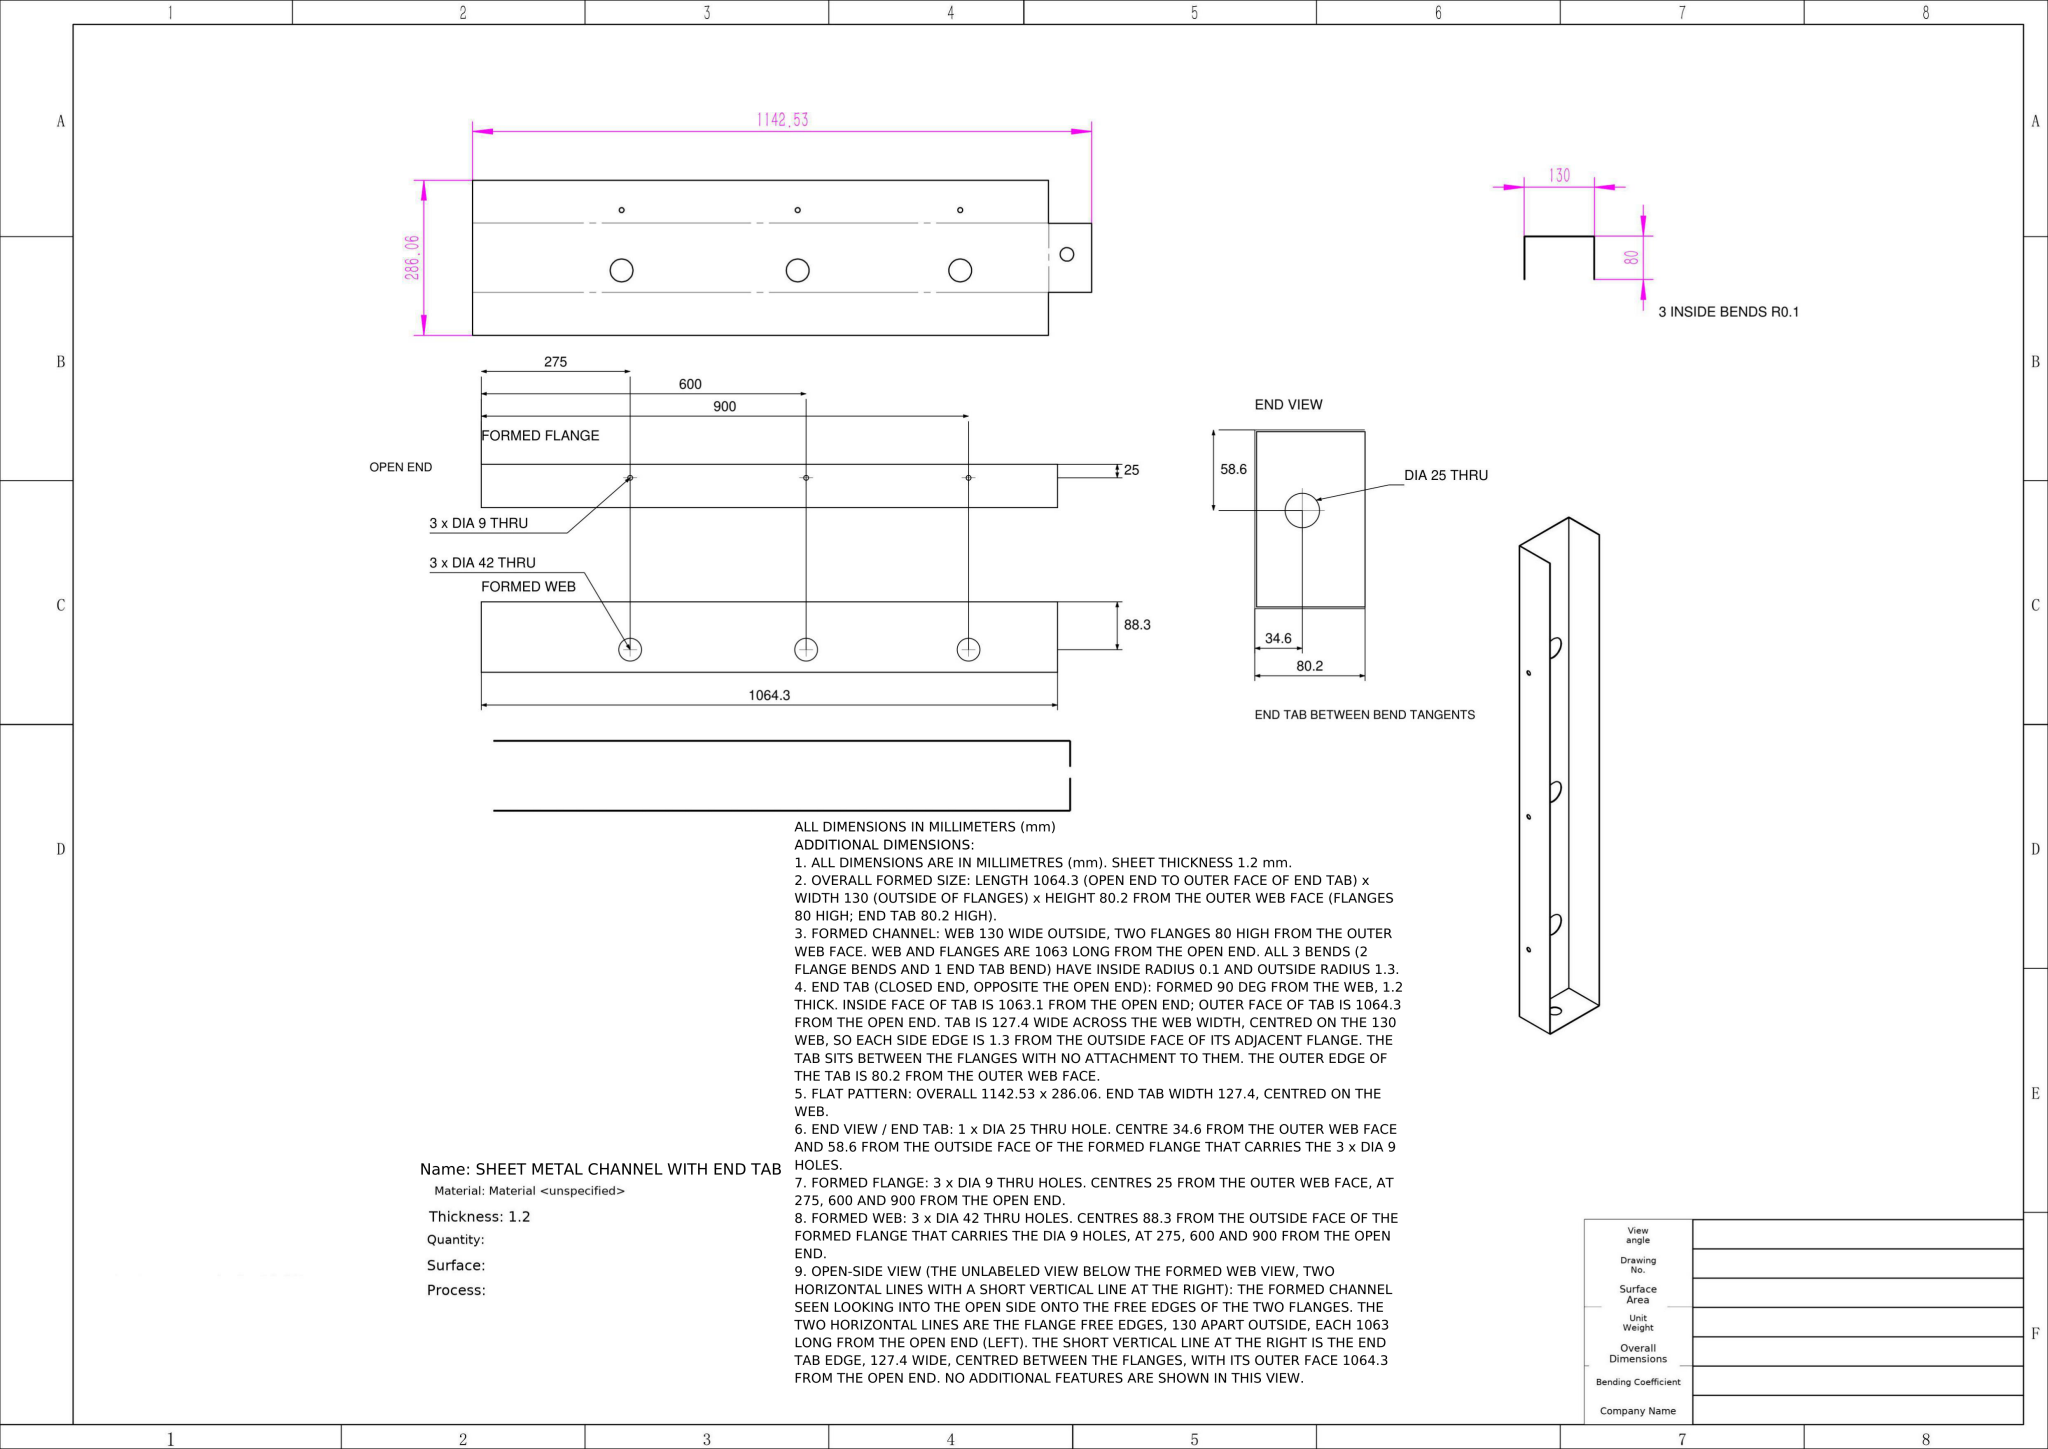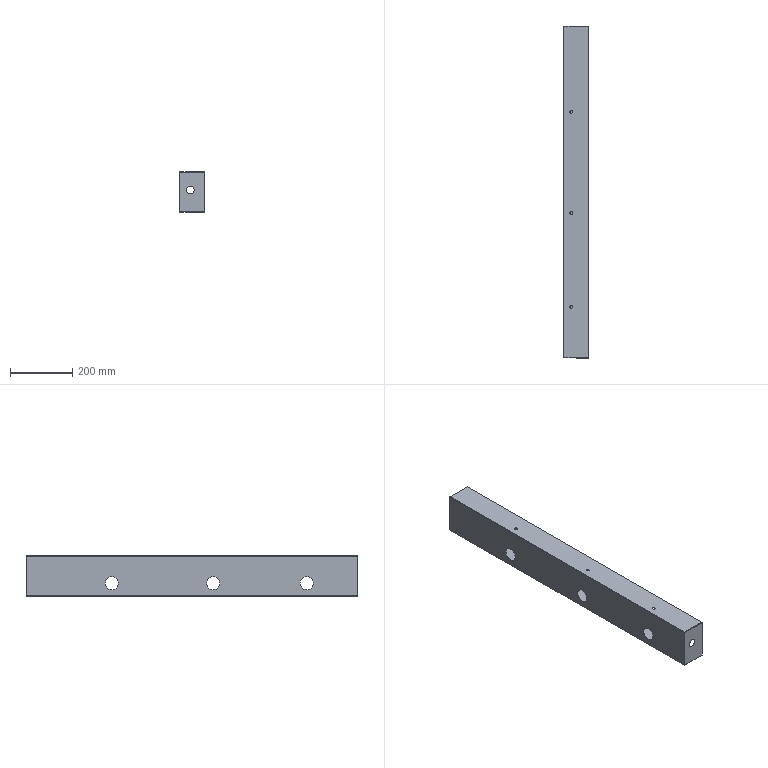Part | NX | mm | 1 solid | 44 faces | box 80.2 x 1064.3 x 130 mm | volume 372521 mm3 | plane 24 | cylinder 20 | commonest cylinder face diameters 9 x6 42 x6 2.6 x3 0.2 x3 25 x2